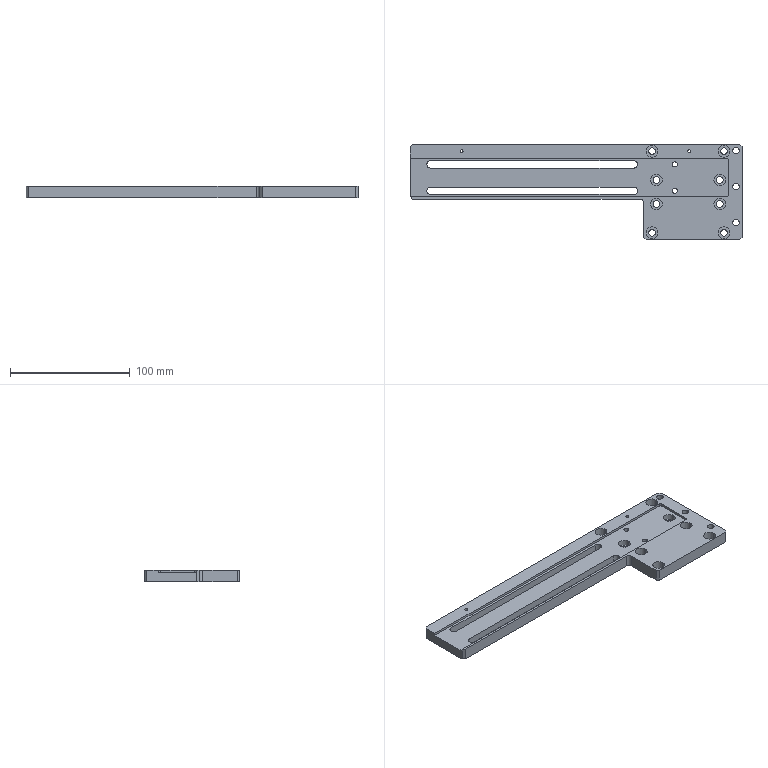Component | SolidWorks | MTCTV2104DJ006-007-0000AdjustableAssembly-1_MTCTV2104DJ006-000-0043SlidePlate-1 | 1 solid | 97 faces | box 277 x 80 x 10 mm | volume 114771 mm3 | cylinder 63 | plane 32 | cone 2 | commonest cylinder face diameters 9.8 x22 5.5 x22 6 x7 4.2 x6 2.5 x4 4 x2
build123d program:
from build123d import *

# Parameters (mm, degrees)
SKETCH1_W                                           = 277
SKETCH1_H                                           = 66
BOSS_EXTRUDE1_DEPTH                                 = 10
SKETCH10_W                                          = 277
SKETCH10_H                                          = 7
BOSS_EXTRUDE2_DEPTH                                 = 10
HOLE_SIZE_TYPE_OF_HEXAGON_SOCKET_HEAD_C_D           = 5.5
HOLE_SIZE_TYPE_OF_HEXAGON_SOCKET_HEAD_C_CBORE_D     = 9.8
HOLE_SIZE_TYPE_OF_HEXAGON_SOCKET_HEAD_C_CBORE_DEPTH = 7
M3_TAPPED_HOLE1_D                                   = 2.5
SKETCH11_W                                          = 277
SKETCH11_H                                          = 32
CUT_EXTRUDE1_DEPTH                                  = 2
M5_TAPPED_HOLE1_D                                   = 4.2
CUT_EXTRUDE2_DEPTH                                  = 145.382
SKETCH17_W                                          = 11
SKETCH17_H                                          = 32
BOSS_EXTRUDE3_DEPTH                                 = 2
HOLE_SIZE_TYPE_OF_HEXAGON_SOCKET_HE_2_D             = 5.5
HOLE_SIZE_TYPE_OF_HEXAGON_SOCKET_HE_2_CBORE_D       = 9.8
HOLE_SIZE_TYPE_OF_HEXAGON_SOCKET_HE_2_CBORE_DEPTH   = 6
M5_TAPPED_HOLE2_D                                   = 4.2
M5_TAPPED_HOLE2_DEPTH                               = 14
M5_TAPPED_HOLE2_TIP                                 = 1.262
SKETCH22_W                                          = 195
SKETCH22_H                                          = 34
CUT_EXTRUDE3_DEPTH                                  = 145.507
FILLET1_R                                           = 3
FILLET2_R                                           = 2
CHAMFER1_SIZE                                       = 2


with BuildPart() as part:
    # Sketch1 → Boss-Extrude1 (new body)
    with BuildSketch(Plane(origin=(0, 0, 0), x_dir=(0, 0, -1), z_dir=(1, 0, 0))):
        Rectangle(SKETCH1_W, SKETCH1_H)
    extrude(amount=BOSS_EXTRUDE1_DEPTH)

    # Sketch10 → Boss-Extrude2 (add, through all)
    with BuildSketch(Plane(origin=(10, 0, 0), x_dir=(0, 0, -1), z_dir=(1, 0, 0))):
        with Locations((0, 36.5)):
            Rectangle(SKETCH10_W, SKETCH10_H)
        with Locations((0, -36.5)):
            Rectangle(SKETCH10_W, SKETCH10_H)
    extrude(amount=-BOSS_EXTRUDE2_DEPTH)

    # Hole Size _Type of Hexagon Socket Head C (through all)
    with Locations(Plane(origin=(10, 0, 0), x_dir=(0, 0, 1), z_dir=(1, 0, 0))):
        with Locations((-123.5, -34), (-123.5, 34), (-63.5, 34), (-63.5, -34), (-120, -10), (-120, 10), (-67, 10), (-67, -10)):
            CounterBoreHole(HOLE_SIZE_TYPE_OF_HEXAGON_SOCKET_HEAD_C_D / 2, HOLE_SIZE_TYPE_OF_HEXAGON_SOCKET_HEAD_C_CBORE_D / 2, HOLE_SIZE_TYPE_OF_HEXAGON_SOCKET_HEAD_C_CBORE_DEPTH)

    # M3 Tapped Hole1 (through all)
    with Locations(Plane.ZY):
        with Locations((-94.5, 34), (95.5, 34)):
            Hole(M3_TAPPED_HOLE1_D / 2)

    # Sketch11 → Cut-Extrude1 (cut)
    with BuildSketch(Plane(origin=(10, 0, 0), x_dir=(0, 0, -1), z_dir=(1, 0, 0))):
        with Locations((0, 12)):
            Rectangle(SKETCH11_W, SKETCH11_H)
    extrude(amount=-CUT_EXTRUDE1_DEPTH, mode=Mode.SUBTRACT)

    # M5 Tapped Hole1 (through all)
    with Locations(Plane(origin=(8, 0, 0), x_dir=(0, 0, -1), z_dir=(1, 0, 0))):
        with Locations((82.5, 23), (82.5, 1)):
            Hole(M5_TAPPED_HOLE1_D / 2)

    # Sketch14 → Cut-Extrude2 (cut, through all)
    with BuildSketch(Plane(origin=(8, 0, 0), x_dir=(0, 0, -1), z_dir=(1, 0, 0))):
        with BuildLine():
            Line((-121.5, 26), (48.5, 26))
            ThreePointArc((48.5, 26), (51.5, 23), (48.5, 20))
            Line((48.5, 20), (-121.5, 20))
            ThreePointArc((-121.5, 20), (-124.5, 23), (-121.5, 26))
        make_face()
        with BuildLine():
            Line((-121.5, 4), (48.5, 4))
            ThreePointArc((48.5, 4), (51.5, 1), (48.5, -2))
            Line((48.5, -2), (-121.5, -2))
            ThreePointArc((-121.5, -2), (-124.5, 1), (-121.5, 4))
        make_face()
    extrude(amount=-CUT_EXTRUDE2_DEPTH, mode=Mode.SUBTRACT)

    # Sketch17 → Boss-Extrude3 (add)
    with BuildSketch(Plane(origin=(8, 0, 0), x_dir=(0, 0, -1), z_dir=(1, 0, 0))):
        with Locations((133, 12)):
            Rectangle(SKETCH17_W, SKETCH17_H)
    extrude(amount=BOSS_EXTRUDE3_DEPTH)

    # Hole Size _Type of Hexagon Socket He 2 (through all)
    with Locations(Plane.ZY):
        with Locations((-133.5, 34.5), (-133.5, 4.5), (-133.5, -25.5)):
            CounterBoreHole(HOLE_SIZE_TYPE_OF_HEXAGON_SOCKET_HE_2_D / 2, HOLE_SIZE_TYPE_OF_HEXAGON_SOCKET_HE_2_CBORE_D / 2, HOLE_SIZE_TYPE_OF_HEXAGON_SOCKET_HE_2_CBORE_DEPTH)

    # M5 Tapped Hole2
    with Locations(Plane(origin=(0, 40, 0), x_dir=(1, 0, 0), z_dir=(0, 1, 0))):
        with Locations((5, 88.5)):
            Hole(M5_TAPPED_HOLE2_D / 2, depth=M5_TAPPED_HOLE2_DEPTH)
            with Locations((0, 0, -(M5_TAPPED_HOLE2_DEPTH + M5_TAPPED_HOLE2_TIP / 2))):  # 118° drill point
                Cone(0, M5_TAPPED_HOLE2_D / 2, M5_TAPPED_HOLE2_TIP, mode=Mode.SUBTRACT)

    # Sketch22 → Cut-Extrude3 (cut, through all)
    with BuildSketch(Plane(origin=(10, 0, 0), x_dir=(0, 0, -1), z_dir=(1, 0, 0))):
        with Locations((-41, -23)):
            Rectangle(SKETCH22_W, SKETCH22_H)
    extrude(amount=-CUT_EXTRUDE3_DEPTH, mode=Mode.SUBTRACT)

    # Fillet1
    fillet1_edges = [part.edges().sort_by_distance(p)[0] for p in [
        (5, -6, -56.5),
    ]]
    fillet(fillet1_edges, radius=FILLET1_R)

    # Fillet2
    fillet2_edges = [part.edges().sort_by_distance(p)[0] for p in [
        (9, 28, -127.5),
        (9, -4, -127.5),
    ]]
    fillet(fillet2_edges, radius=FILLET2_R)

    # Chamfer1
    chamfer1_edges = [part.edges().sort_by_distance(p)[0] for p in [
        (5, 40, 138.5),
        (5, 40, -138.5),
        (5, -6, 138.5),
        (5, -40, -56.5),
        (5, -40, -138.5),
    ]]
    chamfer(chamfer1_edges, length=CHAMFER1_SIZE)


solid = part.part

# Placed as in the assembly
solid = solid.moved(Location((-78.702, 17.781, 171.447), (0, -90, 0)))